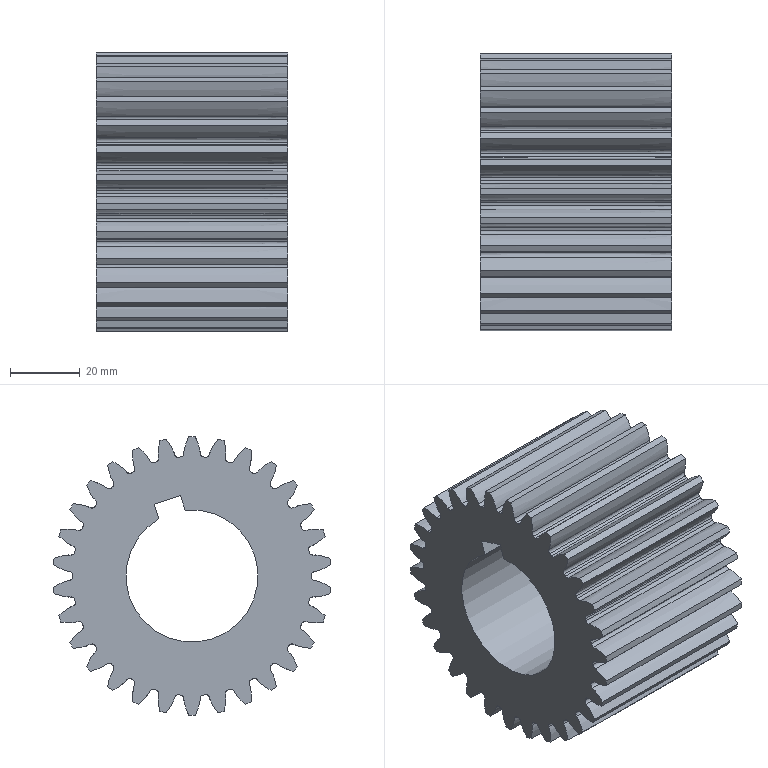Component | NX | CHUANDONGZHOUXIAOCHILUN | 1 solid | 186 faces | volume 176204 mm3 | other 150 | cylinder 31 | plane 5 | commonest cylinder face diameters 68.75 x30 38 x1